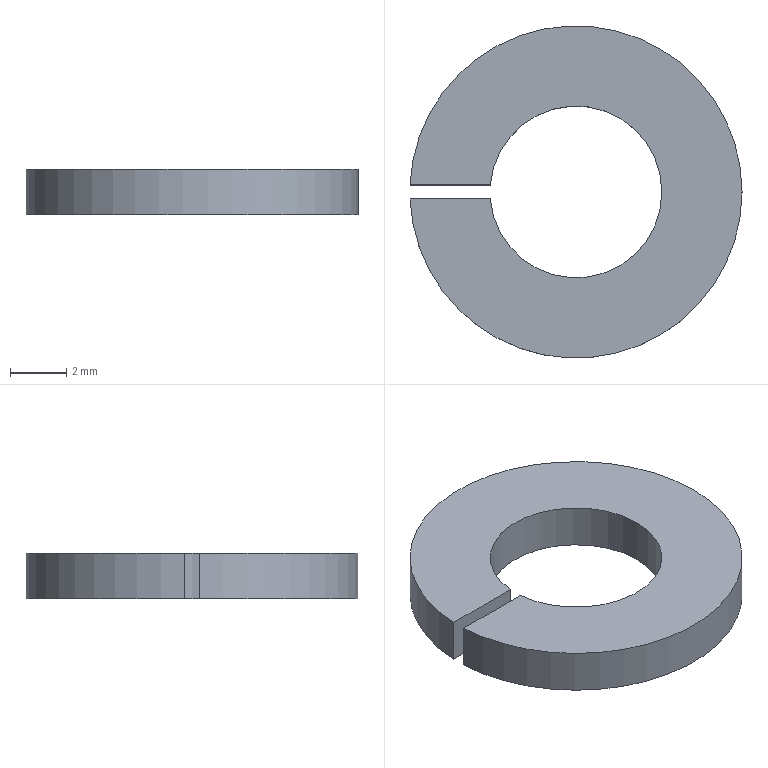Component | SolidWorks | ScrewM6-L20AndSpringWasherAssembly-1_SpringWasherTBN41-6(YIHEDA)-1 | 1 solid | 6 faces | box 11.79 x 11.8 x 1.6 mm | volume 126 mm3 | plane 4 | cylinder 2 | commonest cylinder face diameters 11.8 x1 6.1 x1
STEP:
#1=CARTESIAN_POINT('',(2.144,0.5715,10.201));
#2=VERTEX_POINT('',#1);
#3=CARTESIAN_POINT('',(2.144,0.5912,10.201));
#4=VERTEX_POINT('',#3);
#5=CARTESIAN_POINT('',(2.376,0.5813,10.201));
#6=DIRECTION('',(0.,0.,1.));
#7=DIRECTION('',(1.,0.,0.));
#8=AXIS2_PLACEMENT_3D('',#5,#6,#7);
#9=CIRCLE('',#8,0.2323);
#10=EDGE_CURVE('',#2,#4,#9,.T.);
#11=ORIENTED_EDGE('',*,*,#10,.T.);
#12=CARTESIAN_POINT('',(2.144,0.5912,10.264));
#13=VERTEX_POINT('',#12);
#14=CARTESIAN_POINT('',(2.144,0.5912,10.264));
#15=DIRECTION('',(0.,0.,-1.));
#16=VECTOR('',#15,39.37);
#17=LINE('',#14,#16);
#18=EDGE_CURVE('',#13,#4,#17,.T.);
#19=ORIENTED_EDGE('',*,*,#18,.F.);
#20=CARTESIAN_POINT('',(2.144,0.5715,10.264));
#21=VERTEX_POINT('',#20);
#22=CARTESIAN_POINT('',(2.376,0.5813,10.264));
#23=DIRECTION('',(0.,0.,1.));
#24=DIRECTION('',(1.,0.,0.));
#25=AXIS2_PLACEMENT_3D('',#22,#23,#24);
#26=CIRCLE('',#25,0.2323);
#27=EDGE_CURVE('',#21,#13,#26,.T.);
#28=ORIENTED_EDGE('',*,*,#27,.F.);
#29=CARTESIAN_POINT('',(2.144,0.5715,10.264));
#30=DIRECTION('',(0.,0.,-1.));
#31=VECTOR('',#30,39.37);
#32=LINE('',#29,#31);
#33=EDGE_CURVE('',#21,#2,#32,.T.);
#34=ORIENTED_EDGE('',*,*,#33,.T.);
#35=EDGE_LOOP('',(#11,#19,#28,#34));
#36=FACE_OUTER_BOUND('',#35,.T.);
#37=CARTESIAN_POINT('',(2.376,0.5813,10.264));
#38=DIRECTION('',(0.,0.,1.));
#39=DIRECTION('',(-1.,0.,0.));
#40=AXIS2_PLACEMENT_3D('',#37,#38,#39);
#41=CYLINDRICAL_SURFACE('',#40,0.2323);
#42=ADVANCED_FACE('',(#36),#41,.T.);
#43=ORIENTED_EDGE('',*,*,#27,.T.);
#44=CARTESIAN_POINT('',(2.256,0.5912,10.264));
#45=VERTEX_POINT('',#44);
#46=CARTESIAN_POINT('',(2.144,0.5912,10.264));
#47=DIRECTION('',(1.,0.,0.));
#48=VECTOR('',#47,39.37);
#49=LINE('',#46,#48);
#50=EDGE_CURVE('',#13,#45,#49,.T.);
#51=ORIENTED_EDGE('',*,*,#50,.T.);
#52=CARTESIAN_POINT('',(2.256,0.5715,10.264));
#53=VERTEX_POINT('',#52);
#54=CARTESIAN_POINT('',(2.376,0.5813,10.264));
#55=DIRECTION('',(0.,0.,1.));
#56=DIRECTION('',(1.,0.,0.));
#57=AXIS2_PLACEMENT_3D('',#54,#55,#56);
#58=CIRCLE('',#57,0.1201);
#59=EDGE_CURVE('',#53,#45,#58,.T.);
#60=ORIENTED_EDGE('',*,*,#59,.F.);
#61=CARTESIAN_POINT('',(2.256,0.5715,10.264));
#62=DIRECTION('',(-1.,0.,0.));
#63=VECTOR('',#62,39.37);
#64=LINE('',#61,#63);
#65=EDGE_CURVE('',#53,#21,#64,.T.);
#66=ORIENTED_EDGE('',*,*,#65,.T.);
#67=EDGE_LOOP('',(#43,#51,#60,#66));
#68=FACE_OUTER_BOUND('',#67,.T.);
#69=CARTESIAN_POINT('',(2.376,0.5813,10.264));
#70=DIRECTION('',(0.,0.,1.));
#71=DIRECTION('',(1.,0.,0.));
#72=AXIS2_PLACEMENT_3D('',#69,#70,#71);
#73=PLANE('',#72);
#74=ADVANCED_FACE('',(#68),#73,.T.);
#75=CARTESIAN_POINT('',(2.256,0.5912,10.201));
#76=VERTEX_POINT('',#75);
#77=CARTESIAN_POINT('',(2.144,0.5912,10.201));
#78=DIRECTION('',(1.,0.,0.));
#79=VECTOR('',#78,39.37);
#80=LINE('',#77,#79);
#81=EDGE_CURVE('',#4,#76,#80,.T.);
#82=ORIENTED_EDGE('',*,*,#81,.T.);
#83=CARTESIAN_POINT('',(2.256,0.5912,10.264));
#84=DIRECTION('',(0.,0.,-1.));
#85=VECTOR('',#84,39.37);
#86=LINE('',#83,#85);
#87=EDGE_CURVE('',#45,#76,#86,.T.);
#88=ORIENTED_EDGE('',*,*,#87,.F.);
#89=ORIENTED_EDGE('',*,*,#50,.F.);
#90=ORIENTED_EDGE('',*,*,#18,.T.);
#91=EDGE_LOOP('',(#82,#88,#89,#90));
#92=FACE_OUTER_BOUND('',#91,.T.);
#93=CARTESIAN_POINT('',(2.144,0.5912,10.264));
#94=DIRECTION('',(0.,1.,0.));
#95=DIRECTION('',(1.,0.,0.));
#96=AXIS2_PLACEMENT_3D('',#93,#94,#95);
#97=PLANE('',#96);
#98=ADVANCED_FACE('',(#92),#97,.F.);
#99=CARTESIAN_POINT('',(2.256,0.5715,10.201));
#100=VERTEX_POINT('',#99);
#101=CARTESIAN_POINT('',(2.376,0.5813,10.201));
#102=DIRECTION('',(0.,0.,1.));
#103=DIRECTION('',(1.,0.,0.));
#104=AXIS2_PLACEMENT_3D('',#101,#102,#103);
#105=CIRCLE('',#104,0.1201);
#106=EDGE_CURVE('',#100,#76,#105,.T.);
#107=ORIENTED_EDGE('',*,*,#106,.F.);
#108=CARTESIAN_POINT('',(2.256,0.5715,10.264));
#109=DIRECTION('',(0.,0.,-1.));
#110=VECTOR('',#109,39.37);
#111=LINE('',#108,#110);
#112=EDGE_CURVE('',#53,#100,#111,.T.);
#113=ORIENTED_EDGE('',*,*,#112,.F.);
#114=ORIENTED_EDGE('',*,*,#59,.T.);
#115=ORIENTED_EDGE('',*,*,#87,.T.);
#116=EDGE_LOOP('',(#107,#113,#114,#115));
#117=FACE_OUTER_BOUND('',#116,.T.);
#118=CARTESIAN_POINT('',(2.376,0.5813,10.264));
#119=DIRECTION('',(0.,0.,1.));
#120=DIRECTION('',(-1.,0.,0.));
#121=AXIS2_PLACEMENT_3D('',#118,#119,#120);
#122=CYLINDRICAL_SURFACE('',#121,0.1201);
#123=ADVANCED_FACE('',(#117),#122,.F.);
#124=ORIENTED_EDGE('',*,*,#10,.F.);
#125=CARTESIAN_POINT('',(2.256,0.5715,10.201));
#126=DIRECTION('',(-1.,0.,0.));
#127=VECTOR('',#126,39.37);
#128=LINE('',#125,#127);
#129=EDGE_CURVE('',#100,#2,#128,.T.);
#130=ORIENTED_EDGE('',*,*,#129,.F.);
#131=ORIENTED_EDGE('',*,*,#106,.T.);
#132=ORIENTED_EDGE('',*,*,#81,.F.);
#133=EDGE_LOOP('',(#124,#130,#131,#132));
#134=FACE_OUTER_BOUND('',#133,.T.);
#135=CARTESIAN_POINT('',(2.376,0.5813,10.201));
#136=DIRECTION('',(0.,0.,1.));
#137=DIRECTION('',(1.,0.,0.));
#138=AXIS2_PLACEMENT_3D('',#135,#136,#137);
#139=PLANE('',#138);
#140=ADVANCED_FACE('',(#134),#139,.F.);
#141=ORIENTED_EDGE('',*,*,#129,.T.);
#142=ORIENTED_EDGE('',*,*,#33,.F.);
#143=ORIENTED_EDGE('',*,*,#65,.F.);
#144=ORIENTED_EDGE('',*,*,#112,.T.);
#145=EDGE_LOOP('',(#141,#142,#143,#144));
#146=FACE_OUTER_BOUND('',#145,.T.);
#147=CARTESIAN_POINT('',(2.256,0.5715,10.264));
#148=DIRECTION('',(0.,-1.,0.));
#149=DIRECTION('',(0.,0.,-1.));
#150=AXIS2_PLACEMENT_3D('',#147,#148,#149);
#151=PLANE('',#150);
#152=ADVANCED_FACE('',(#146),#151,.F.);
#153=CLOSED_SHELL('',(#42,#74,#98,#123,#140,#152));
#154=MANIFOLD_SOLID_BREP('',#153);
#155=CARTESIAN_POINT('',(0.,0.,0.));
#156=DIRECTION('',(0.,0.,1.));
#157=DIRECTION('',(1.,0.,0.));
#158=AXIS2_PLACEMENT_3D('',#155,#156,#157);
#159=(LENGTH_UNIT()NAMED_UNIT(*)SI_UNIT($,.METRE.));
#160=LENGTH_MEASURE_WITH_UNIT(LENGTH_MEASURE(0.0254),#159);
#161=DIMENSIONAL_EXPONENTS(1.,0.,0.,0.,0.,0.,0.);
#162=(CONVERSION_BASED_UNIT('',#160)LENGTH_UNIT()NAMED_UNIT(#161));
#163=UNCERTAINTY_MEASURE_WITH_UNIT(LENGTH_MEASURE(0.00001),#162,'','');
#164=(NAMED_UNIT(*)PLANE_ANGLE_UNIT()SI_UNIT($,.RADIAN.));
#165=(NAMED_UNIT(*)SI_UNIT($,.STERADIAN.)SOLID_ANGLE_UNIT());
#166=(GEOMETRIC_REPRESENTATION_CONTEXT(3)GLOBAL_UNCERTAINTY_ASSIGNED_CONTEXT((#163))GLOBAL_UNIT_ASSIGNED_CONTEXT((#162,#164,#165))REPRESENTATION_CONTEXT('',''));
#167=ADVANCED_BREP_SHAPE_REPRESENTATION('',(#154,#158),#166);
#168=COLOUR_RGB('',0.7922,0.8196,0.9333);
#169=FILL_AREA_STYLE_COLOUR('',#168);
#170=FILL_AREA_STYLE('',(#169));
#171=SURFACE_STYLE_FILL_AREA(#170);
#172=SURFACE_SIDE_STYLE('',(#171));
#173=SURFACE_STYLE_USAGE(.BOTH.,#172);
#174=PRESENTATION_STYLE_ASSIGNMENT((#173));
#175=STYLED_ITEM('',(#174),#154);
#176=PRESENTATION_LAYER_ASSIGNMENT('','',(#175));
#177=(LENGTH_UNIT()NAMED_UNIT(*)SI_UNIT($,.METRE.));
#178=LENGTH_MEASURE_WITH_UNIT(LENGTH_MEASURE(0.0254),#177);
#179=DIMENSIONAL_EXPONENTS(1.,0.,0.,0.,0.,0.,0.);
#180=(CONVERSION_BASED_UNIT('',#178)LENGTH_UNIT()NAMED_UNIT(#179));
#181=UNCERTAINTY_MEASURE_WITH_UNIT(LENGTH_MEASURE(0.00001),#180,'','');
#182=(NAMED_UNIT(*)PLANE_ANGLE_UNIT()SI_UNIT($,.RADIAN.));
#183=(NAMED_UNIT(*)SI_UNIT($,.STERADIAN.)SOLID_ANGLE_UNIT());
#184=(GEOMETRIC_REPRESENTATION_CONTEXT(3)GLOBAL_UNCERTAINTY_ASSIGNED_CONTEXT((#181))GLOBAL_UNIT_ASSIGNED_CONTEXT((#180,#182,#183))REPRESENTATION_CONTEXT('',''));
#185=MECHANICAL_DESIGN_GEOMETRIC_PRESENTATION_REPRESENTATION('',(#175),#184);